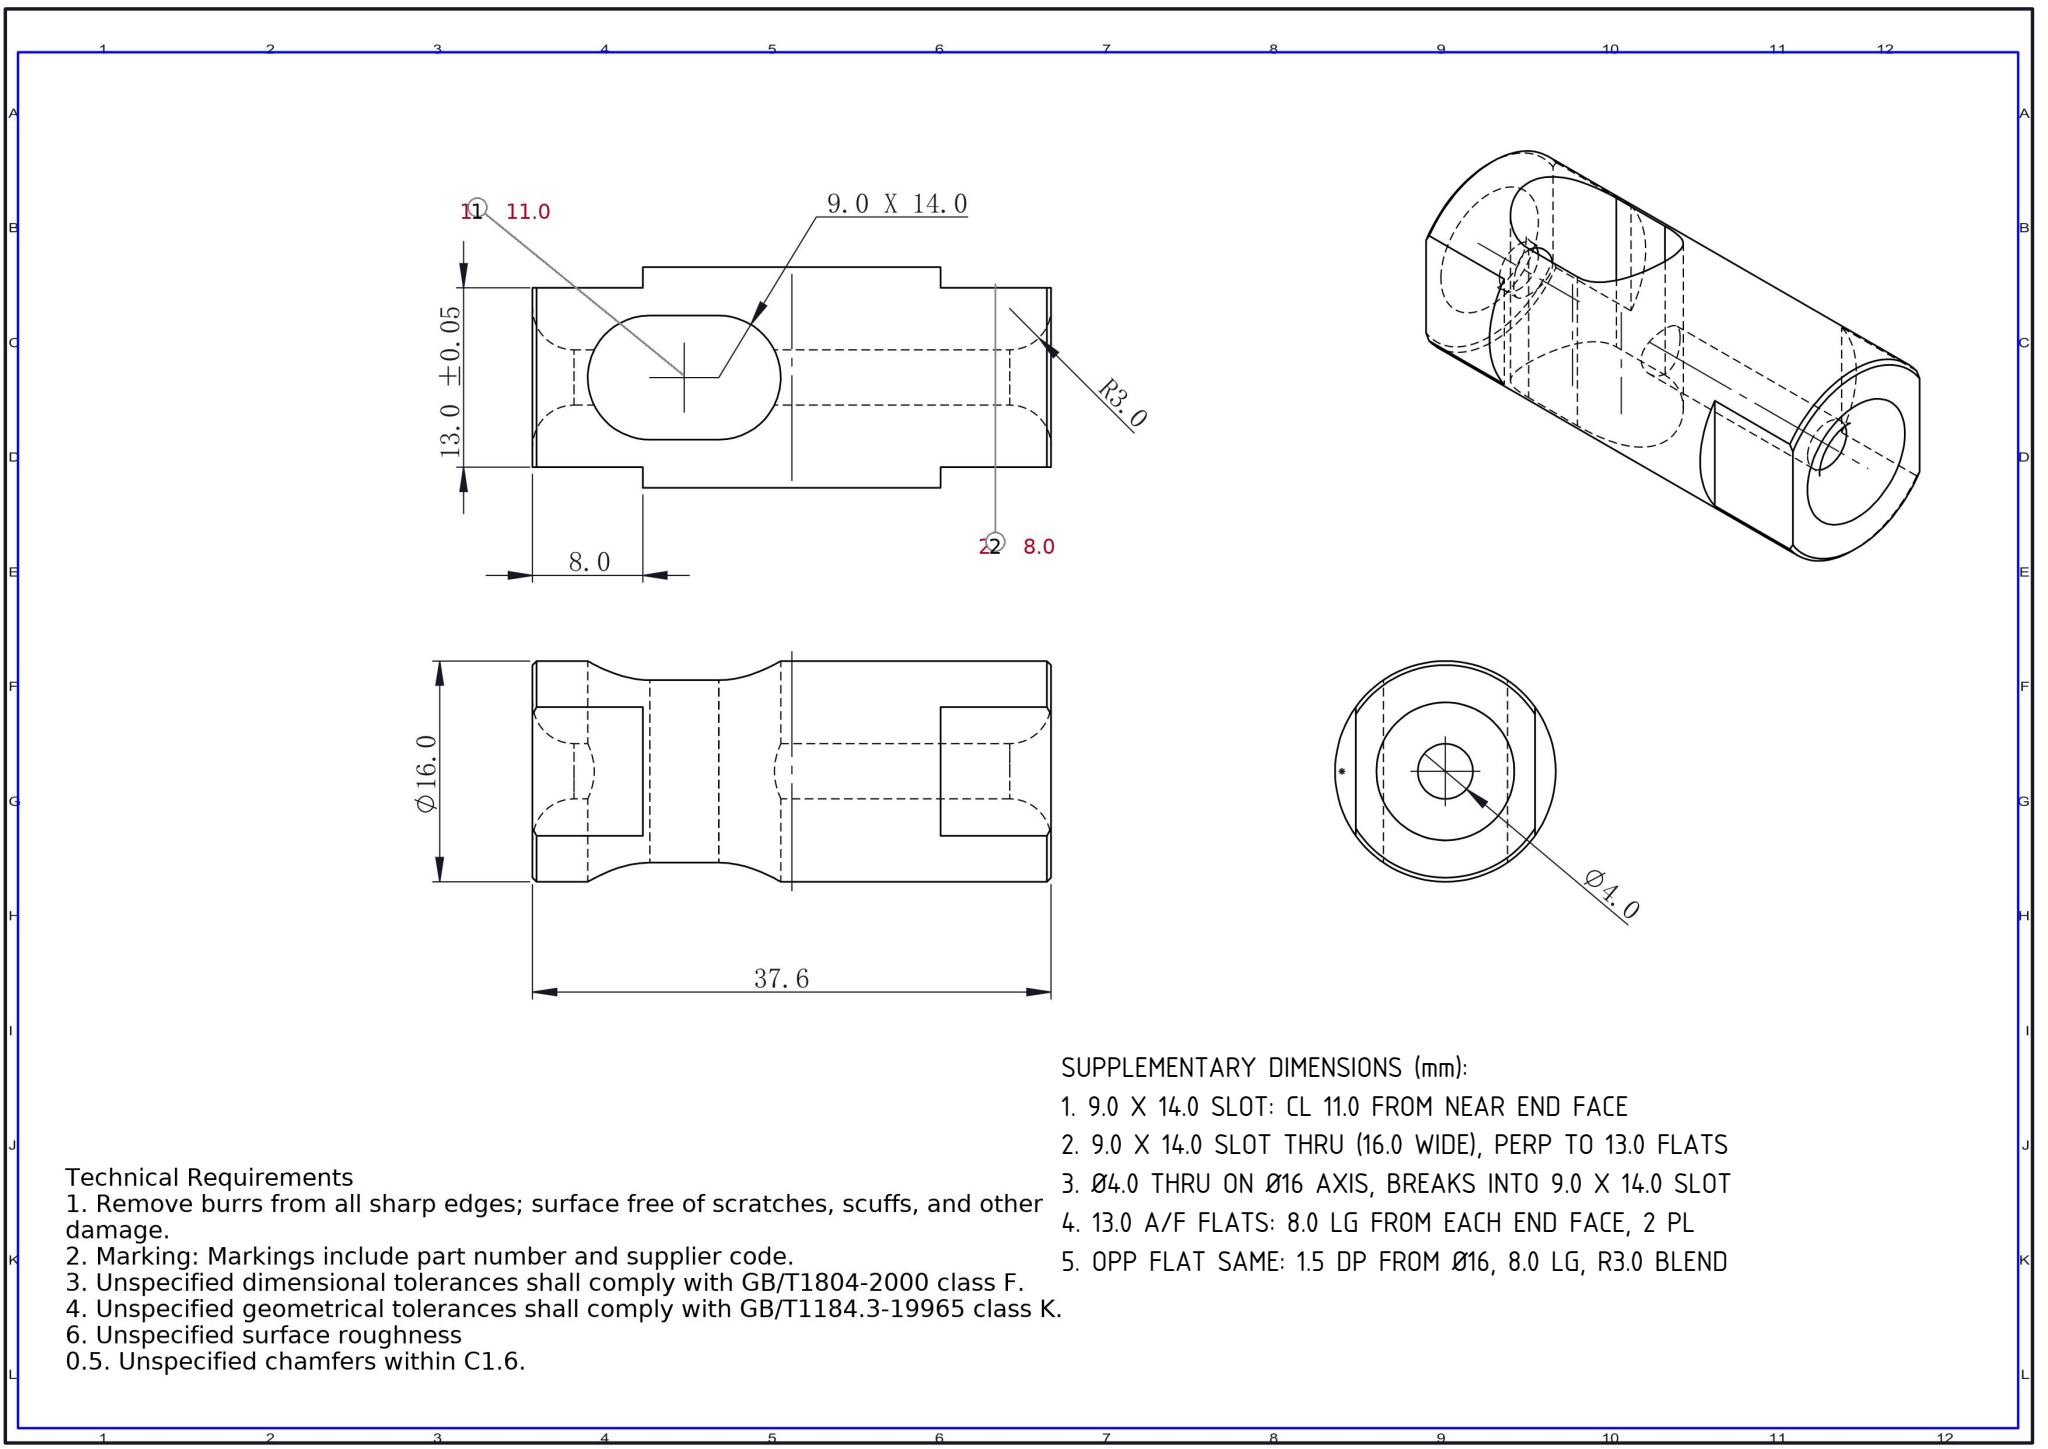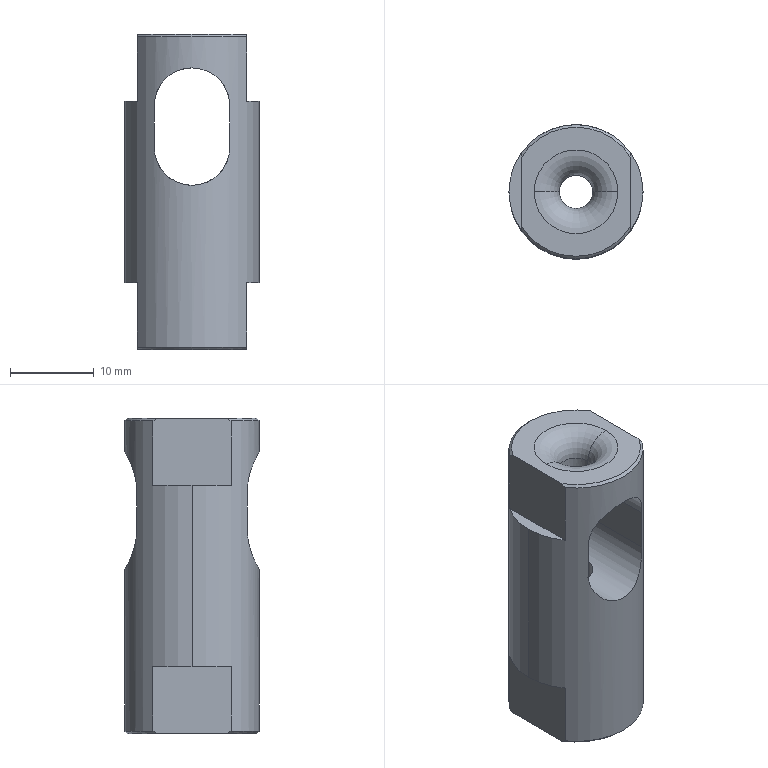Part | SolidWorks | mm | 1 solid | 29 faces | box 16 x 16 x 37.6 mm | volume 5233 mm3 | plane 12 | cylinder 9 | torus 4 | cone 4 | commonest cylinder face diameters 4 x4 9 x3 16 x2
build123d program:
from build123d import *

# Parameters (mm, degrees)
SKETCH1_R           = 8
SKETCH1_R_2         = 2
BOSS_EXTRUDE1_DEPTH = 37.6
CUT_EXTRUDE1_DEPTH  = 20
SKETCH3_OUTSIDE_W   = 26.776
SKETCH3_OUTSIDE_H   = 26.776
SKETCH3_OUTSIDE_W_2 = 13
SKETCH3_OUTSIDE_H_2 = 19.15
CUT_EXTRUDE2_DEPTH  = 8
SKETCH4_OUTSIDE_W   = 26.776
SKETCH4_OUTSIDE_H   = 26.776
SKETCH4_OUTSIDE_W_2 = 13
SKETCH4_OUTSIDE_H_2 = 18.37
CUT_EXTRUDE3_DEPTH  = 8
FILLET1_R           = 3
CHAMFER1_SIZE       = 0.3


with BuildPart() as part:
    # Sketch1 → Boss-Extrude1 (new body)
    with BuildSketch(Plane.XY):
        Circle(SKETCH1_R)
        Circle(SKETCH1_R_2, mode=Mode.SUBTRACT)
    extrude(amount=BOSS_EXTRUDE1_DEPTH)

    # Sketch2 → Cut-Extrude1 (cut, symmetric)
    with BuildSketch(Plane(origin=(0, 0, 0), x_dir=(1, 0, 0), z_dir=(0, 1, 0))):
        with BuildLine():
            Line((4.5, -24.1), (4.5, -29.1))
            ThreePointArc((4.5, -29.1), (0, -33.6), (-4.5, -29.1))
            Line((-4.5, -29.1), (-4.5, -24.1))
            ThreePointArc((-4.5, -24.1), (0, -19.6), (4.5, -24.1))
        make_face()
    extrude(amount=CUT_EXTRUDE1_DEPTH, both=True, mode=Mode.SUBTRACT)

    # Sketch3 outside → Cut-Extrude2 (cut)
    with BuildSketch(Plane.XY.offset(37.6)):
        Rectangle(SKETCH3_OUTSIDE_W, SKETCH3_OUTSIDE_H)
        Rectangle(SKETCH3_OUTSIDE_W_2, SKETCH3_OUTSIDE_H_2, mode=Mode.SUBTRACT)
    extrude(amount=-CUT_EXTRUDE2_DEPTH, mode=Mode.SUBTRACT)

    # Sketch4 outside → Cut-Extrude3 (cut)
    with BuildSketch(Plane(origin=(0, 0, 0), x_dir=(-1, 0, 0), z_dir=(0, 0, -1))):
        Rectangle(SKETCH4_OUTSIDE_W, SKETCH4_OUTSIDE_H)
        Rectangle(SKETCH4_OUTSIDE_W_2, SKETCH4_OUTSIDE_H_2, mode=Mode.SUBTRACT)
    extrude(amount=-CUT_EXTRUDE3_DEPTH, mode=Mode.SUBTRACT)

    # Fillet1
    fillet1_edges = [part.edges().sort_by_distance(p)[0] for p in [
        (-2, 0, 0),
        (-2, 0, 37.6),
    ]]
    fillet(fillet1_edges, radius=FILLET1_R)

    # Chamfer1
    chamfer1_edges = [part.edges().sort_by_distance(p)[0] for p in [
        (0, 8, 0),
        (0, -8, 37.6),
        (0, 8, 37.6),
        (0, -8, 0),
    ]]
    chamfer(chamfer1_edges, length=CHAMFER1_SIZE)


solid = part.part